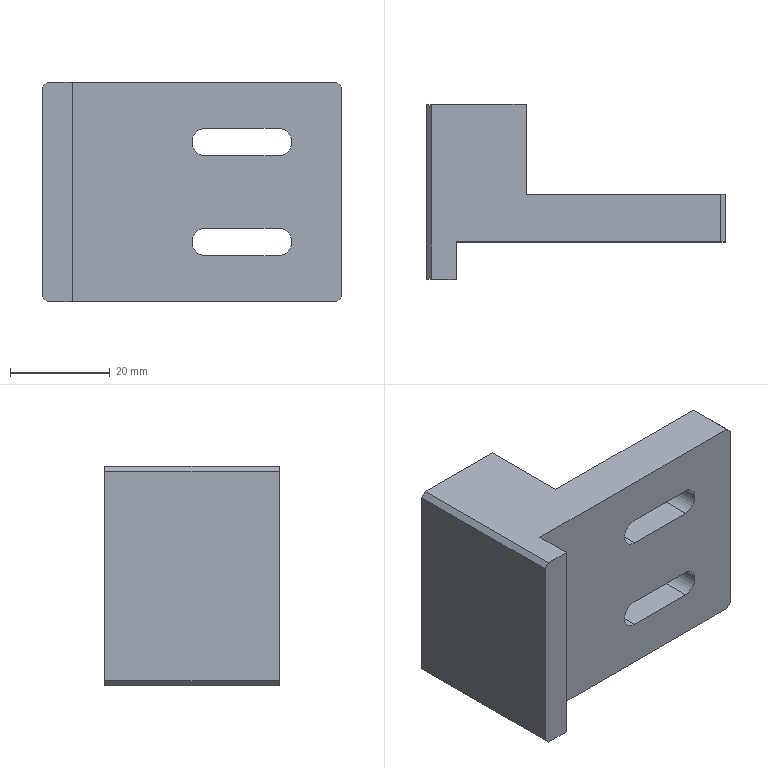CAM job | Mastercam | mm | 12 operations | part box 60 x 35 x 44
1. Facing | 24 - 100 平铣刀
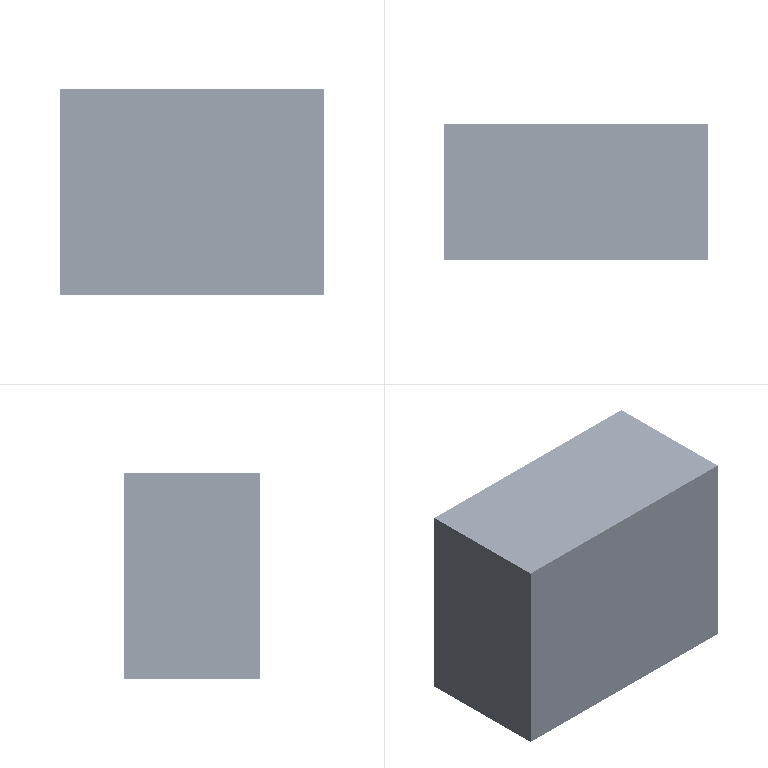2. 2D High Speed (2D Dynamic Mill) | 16 - 16 平铣刀
3. Contour (Ramp) | 16 - 16 平铣刀
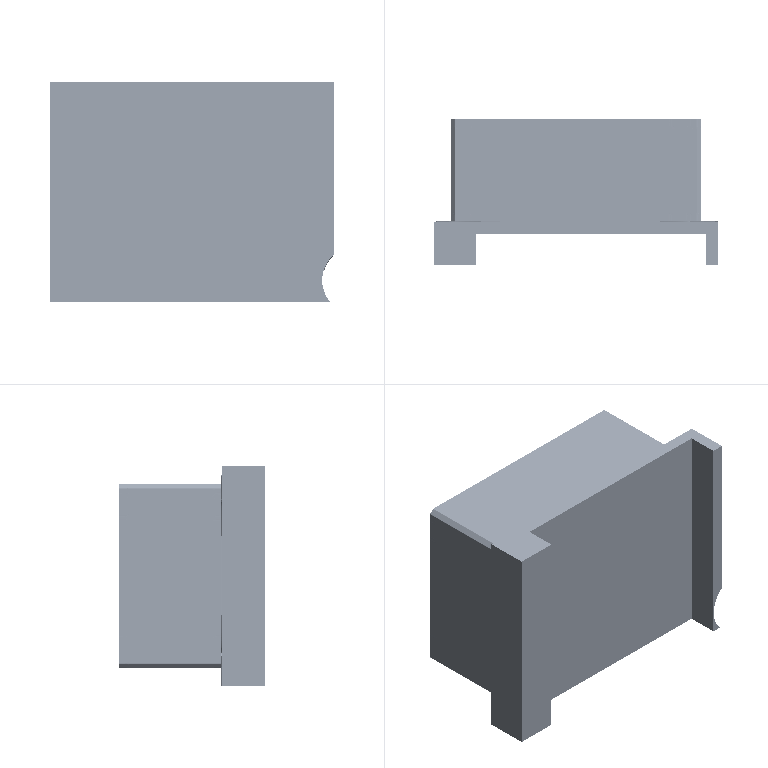4. Contour (2D) | 12 - 12 平铣刀
5. Contour (2D) | 12 - 12 平铣刀
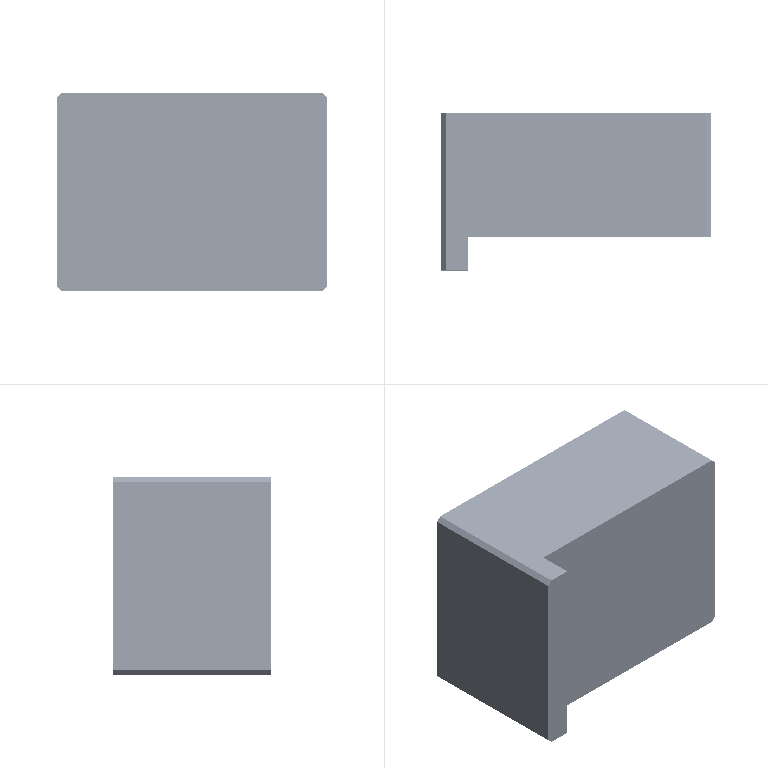6. Contour (Ramp) | 3 - 3 平铣刀
7. Contour (Ramp) | 3 - 3 平铣刀
8. Model Chamfer | 7 - 6 倒角刀
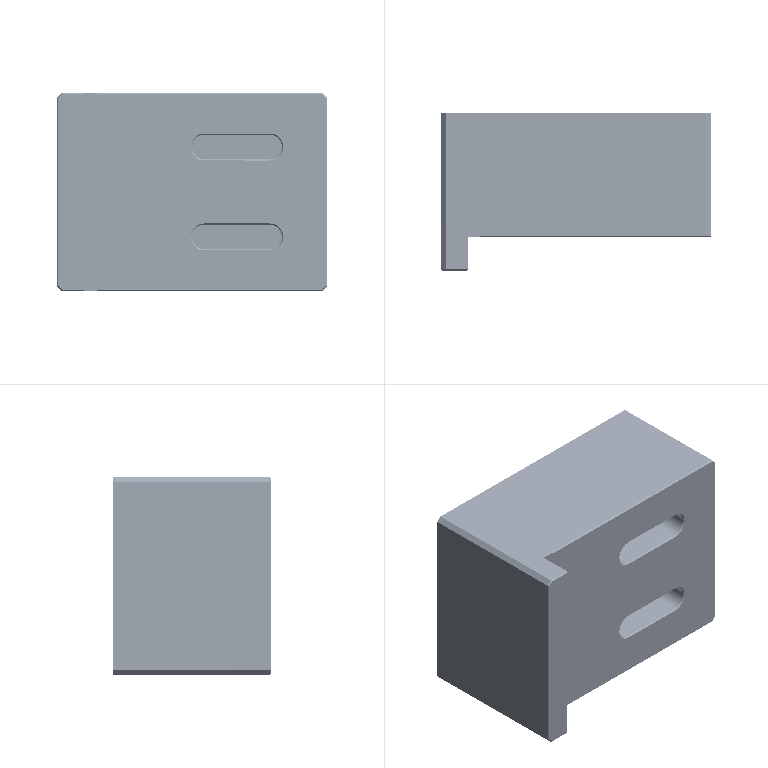9. Facing | 24 - 100 平铣刀
10. Contour (Ramp) | 16 - 16 平铣刀
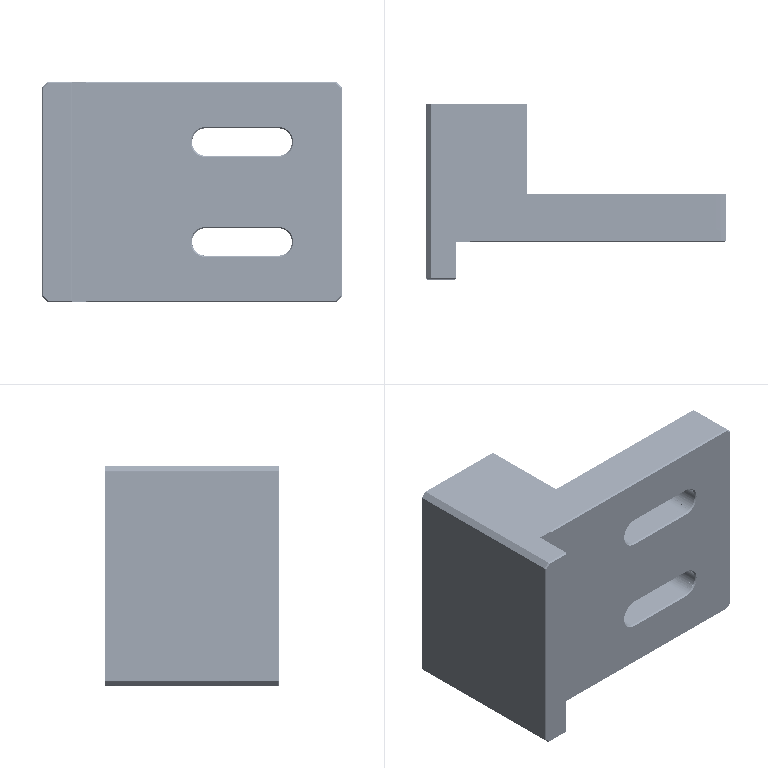11. Contour (2D) | 12 - 12 平铣刀
12. Model Chamfer | 7 - 6 倒角刀